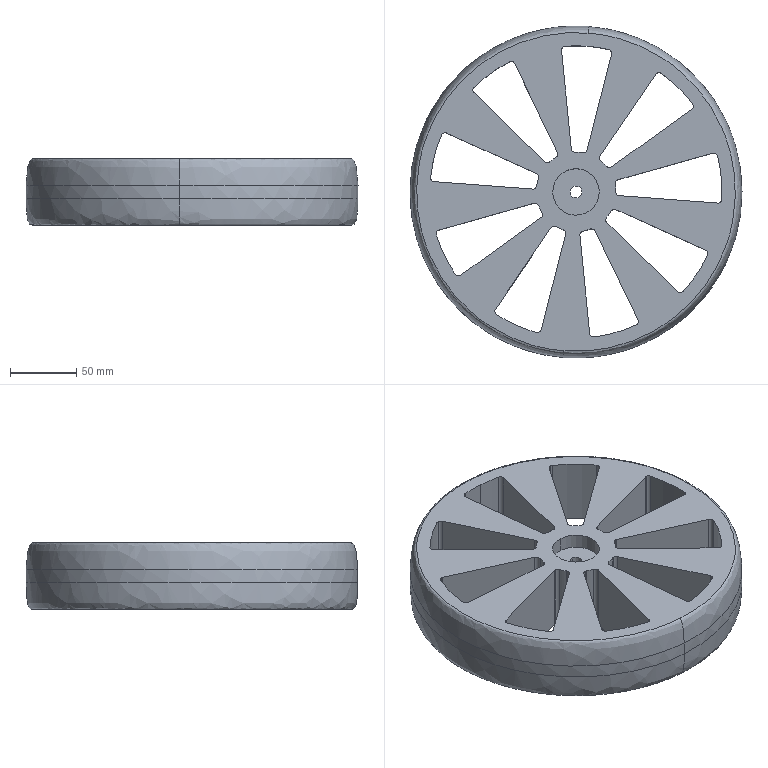Component | SolidWorks | 01-03Wheel-2 | 1 solid | 98 faces | volume 1515719 mm3 | cylinder 72 | plane 22 | spline 4 | commonest cylinder face diameters 6 x44 220 x10 60 x10 9 x2 11 x2 35 x2 250 x2 | material RubberⅠ- 2